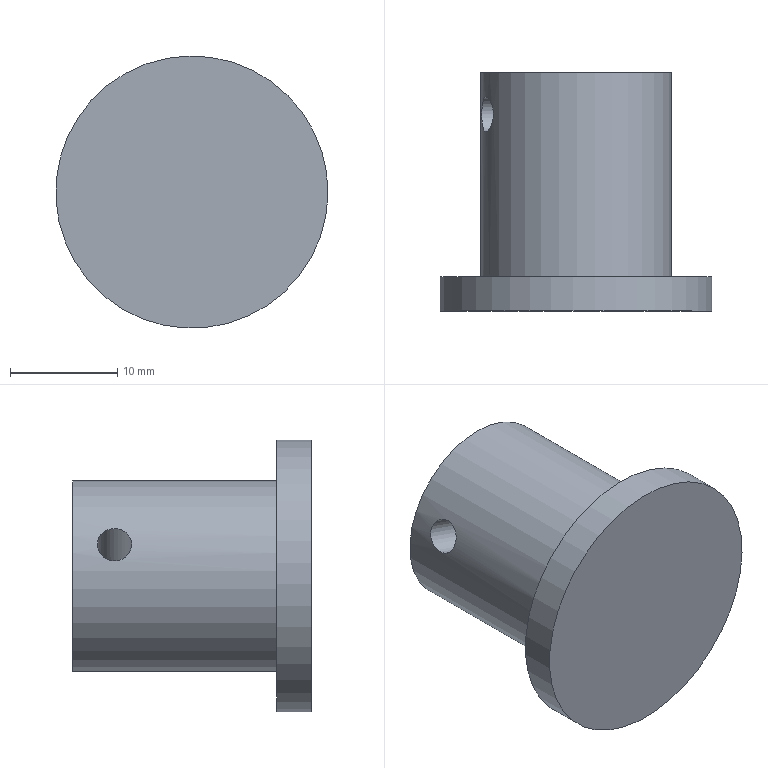Component | NX | PIN_SHAFT | 1 solid | 6 faces | volume 6203 mm3 | cylinder 3 | plane 3 | commonest cylinder face diameters 17.78 x1 25.4 x1 3.2 x1